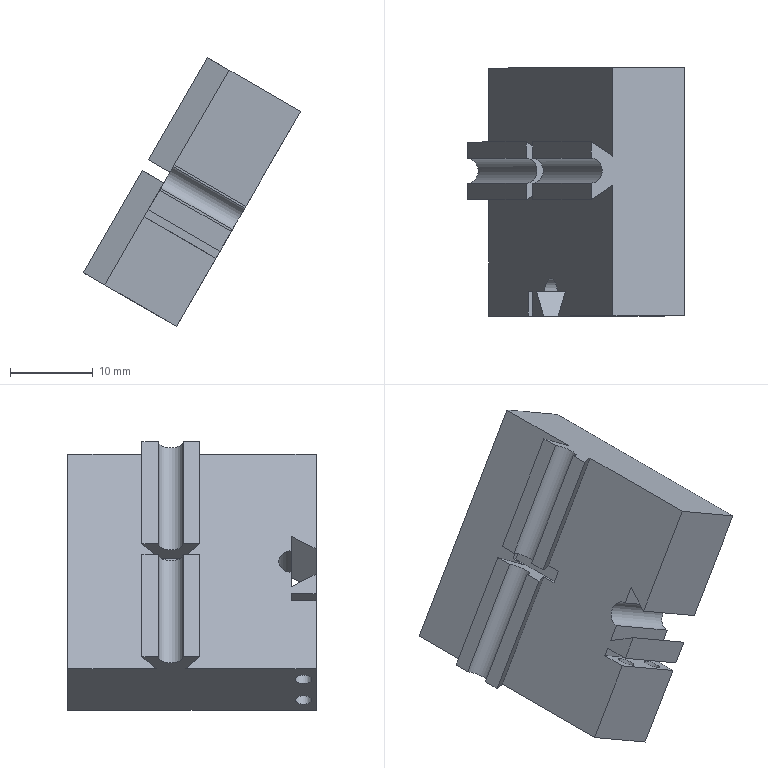Component | SolidWorks | Slider2-2 | 1 solid | 36 faces | box 26.26 x 30 x 32.48 mm | volume 9061 mm3 | plane 29 | cylinder 7 | commonest cylinder face diameters 2 x4 3 x3
build123d program:
from build123d import *

# Parameters (mm, degrees)
BOSS_EXTRUDE1_DEPTH = 10
CUT_EXTRUDE1_REACH  = 37
SKETCH2_R           = 1
BOSS_EXTRUDE3_DEPTH = 15
SKETCH6_W           = 1.5
SKETCH6_H           = 7
CUT_EXTRUDE2_DEPTH  = 3.5


with BuildPart() as part:
    # Sketch1 → Boss-Extrude1 (new body)
    with BuildSketch(Plane(origin=(0, 0, 0), x_dir=(0, 0, -1), z_dir=(1, 0, 0))):
        with BuildLine():
            Line((-15, 15), (15, 15))
            Line((15, 15), (15, -15))
            Line((15, -15), (5.5, -15))
            Line((5.5, -15), (5.5, -12))
            Line((5.5, -12), (4.5, -12))
            Line((4.5, -12), (4.5, -15))
            Line((4.5, -15), (1.768, -15))
            Line((1.768, -15), (3.5, -12))
            Line((3.5, -12), (1.5, -12))
            ThreePointArc((1.5, -12), (0, -10.5), (-1.5, -12))
            Line((-1.5, -12), (-3.5, -12))
            Line((-3.5, -12), (-1.768, -15))
            Line((-1.768, -15), (-15, -15))
            Line((-15, -15), (-15, 15))
        make_face()
    extrude(amount=BOSS_EXTRUDE1_DEPTH)

    # Sketch2 → Cut-Extrude1 (cut, up to next)
    with BuildSketch(Plane(origin=(0, 0, -15), x_dir=(-1, 0, 0), z_dir=(0, 0, -1)), mode=Mode.PRIVATE) as cut_extrude1_sk1:
        with Locations(Location((-2.5, -13.5, 0), (0, 0, 90))):
            Circle(SKETCH2_R)
    cut_extrude1_tool1 = extrude(cut_extrude1_sk1.sketch, amount=-CUT_EXTRUDE1_REACH, mode=Mode.PRIVATE) & part.part
    # Sketch2 → Cut-Extrude1 (cut, up to next)
    with BuildSketch(Plane(origin=(0, 0, -15), x_dir=(-1, 0, 0), z_dir=(0, 0, -1)), mode=Mode.PRIVATE) as cut_extrude1_sk2:
        with Locations((-7.5, -13.5)):
            Circle(SKETCH2_R)
    cut_extrude1_tool2 = extrude(cut_extrude1_sk2.sketch, amount=-CUT_EXTRUDE1_REACH, mode=Mode.PRIVATE) & part.part
    add(cut_extrude1_tool1.solids().sort_by_distance((2.5, -13.5, -15))[0], mode=Mode.SUBTRACT)
    add(cut_extrude1_tool2.solids().sort_by_distance((7.5, -13.5, -15))[0], mode=Mode.SUBTRACT)

    # Sketch5 → Boss-Extrude3 (add, symmetric)
    with BuildSketch(Plane.XY):
        with BuildLine():
            Line((0, 4.322), (0, 0.7864))
            Line((0, 0.7864), (-3, -0.9456))
            Line((-3, -0.9456), (-3, 1.054))
            ThreePointArc((-3, 1.054), (-1.5, 2.554), (-3, 4.054))
            Line((-3, 4.054), (-3, 6.054))
            Line((-3, 6.054), (0, 4.322))
        make_face()
    extrude(amount=BOSS_EXTRUDE3_DEPTH, both=True)

    # Sketch6 → Cut-Extrude2 (cut)
    with BuildSketch(Plane.ZY.offset(3)):
        with Locations((0, 2.554)):
            Rectangle(SKETCH6_W, SKETCH6_H)
    extrude(amount=-CUT_EXTRUDE2_DEPTH, mode=Mode.SUBTRACT)


solid = part.part

# Placed as in the assembly
solid = solid.moved(Location((60.328, 31.006, 121.717), (0, 30, 0)))